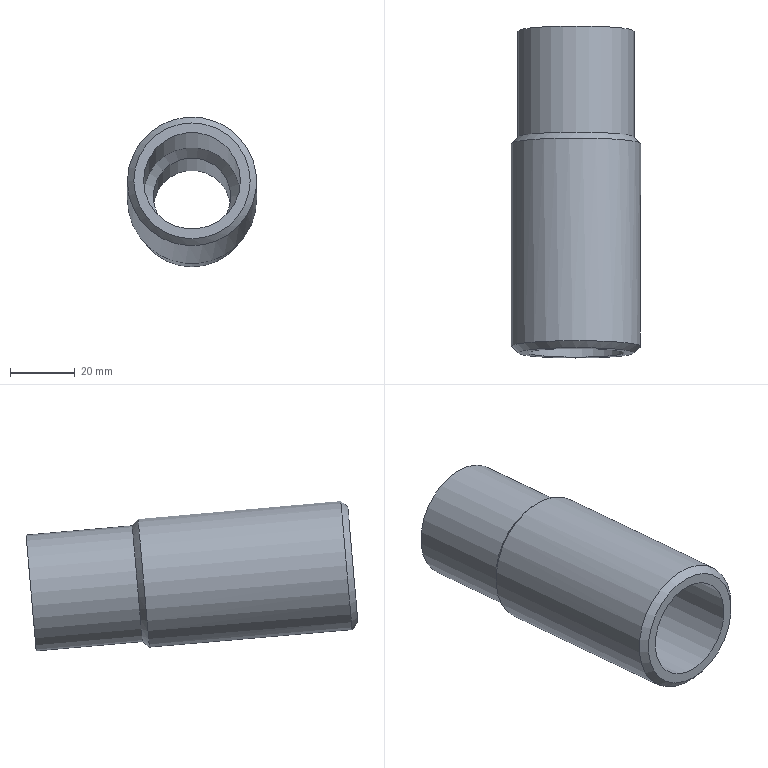Component | NX | HAND_NUT | 1 solid | 9 faces | box 40 x 102.76 x 46.4 mm | volume 58205 mm3 | cylinder 4 | cone 3 | plane 2 | commonest cylinder face diameters 40.005 x1 36.005 x1 30.006 x1 24.008 x1
STEP:
#1=CARTESIAN_POINT('',(0.,0.,0.));
#2=DIRECTION('',(0.,0.,1.));
#3=DIRECTION('',(1.,0.,0.));
#4=AXIS2_PLACEMENT_3D('',#1,#2,#3);
#5=CARTESIAN_POINT('',(323.937,425.208,3.169));
#6=VERTEX_POINT('',#5);
#7=CARTESIAN_POINT('',(335.941,425.208,3.169));
#8=DIRECTION('',(0.,0.9962,-0.08716));
#9=DIRECTION('',(-1.,0.,0.));
#10=AXIS2_PLACEMENT_3D('',#7,#8,#9);
#11=CIRCLE('',#10,12.004);
#12=CARTESIAN_POINT('',(353.941,425.235,3.474));
#13=DIRECTION('',(0.,-0.9962,0.08716));
#14=DIRECTION('',(1.,0.,0.));
#15=AXIS2_PLACEMENT_3D('',#12,#13,#14);
#16=PLANE('',#15);
#17=CARTESIAN_POINT('',(-30.004,-0.3063));
#18=CARTESIAN_POINT('',(-30.004,20.485));
#19=CARTESIAN_POINT('',(-11.998,10.089));
#20=CARTESIAN_POINT('',(6.008,-0.3063));
#21=CARTESIAN_POINT('',(-11.998,-10.702));
#22=CARTESIAN_POINT('',(-30.004,-21.098));
#23=CARTESIAN_POINT('',(-30.004,-0.3063));
#24=(BOUNDED_CURVE()B_SPLINE_CURVE(2,(#17,#18,#19,#20,#21,#22,#23),.UNSPECIFIED.,.T.,.F.)B_SPLINE_CURVE_WITH_KNOTS((1,2,2,2,2,1),(-2.094,0.,2.094,4.189,6.283,8.378),.UNSPECIFIED.)CURVE()GEOMETRIC_REPRESENTATION_ITEM()RATIONAL_B_SPLINE_CURVE((1.,0.5,1.,0.5,1.,0.5,1.))REPRESENTATION_ITEM(''));
#25=(GEOMETRIC_REPRESENTATION_CONTEXT(2)PARAMETRIC_REPRESENTATION_CONTEXT()REPRESENTATION_CONTEXT('',''));
#26=DEFINITIONAL_REPRESENTATION('',(#24),#25);
#27=PCURVE('',#16,#26);
#28=CARTESIAN_POINT('',(335.941,425.208,3.169));
#29=DIRECTION('',(0.,0.9962,-0.08716));
#30=DIRECTION('',(-1.,0.,0.));
#31=AXIS2_PLACEMENT_3D('',#28,#29,#30);
#32=CYLINDRICAL_SURFACE('',#31,12.004);
#33=CARTESIAN_POINT('',(0.,0.));
#34=DIRECTION('',(1.,0.));
#35=VECTOR('',#34,1.);
#36=LINE('',#33,#35);
#37=(GEOMETRIC_REPRESENTATION_CONTEXT(2)PARAMETRIC_REPRESENTATION_CONTEXT()REPRESENTATION_CONTEXT('',''));
#38=DEFINITIONAL_REPRESENTATION('',(#36),#37);
#39=PCURVE('',#32,#38);
#40=SURFACE_CURVE('',#11,(#27,#39),.PCURVE_S1.);
#41=EDGE_CURVE('',#6,#6,#40,.T.);
#42=ORIENTED_EDGE('',*,*,#41,.F.);
#43=EDGE_LOOP('',(#42));
#44=FACE_BOUND('',#43,.T.);
#45=CARTESIAN_POINT('',(317.939,425.208,3.169));
#46=VERTEX_POINT('',#45);
#47=CARTESIAN_POINT('',(335.941,425.208,3.169));
#48=DIRECTION('',(0.,0.9962,-0.08716));
#49=DIRECTION('',(-1.,0.,0.));
#50=AXIS2_PLACEMENT_3D('',#47,#48,#49);
#51=CIRCLE('',#50,18.003);
#52=CARTESIAN_POINT('',(-36.003,-0.3063));
#53=CARTESIAN_POINT('',(-36.003,30.875));
#54=CARTESIAN_POINT('',(-8.999,15.284));
#55=CARTESIAN_POINT('',(18.005,-0.3063));
#56=CARTESIAN_POINT('',(-8.999,-15.897));
#57=CARTESIAN_POINT('',(-36.003,-31.488));
#58=CARTESIAN_POINT('',(-36.003,-0.3063));
#59=(BOUNDED_CURVE()B_SPLINE_CURVE(2,(#52,#53,#54,#55,#56,#57,#58),.UNSPECIFIED.,.T.,.F.)B_SPLINE_CURVE_WITH_KNOTS((1,2,2,2,2,1),(-2.094,0.,2.094,4.189,6.283,8.378),.UNSPECIFIED.)CURVE()GEOMETRIC_REPRESENTATION_ITEM()RATIONAL_B_SPLINE_CURVE((1.,0.5,1.,0.5,1.,0.5,1.))REPRESENTATION_ITEM(''));
#60=(GEOMETRIC_REPRESENTATION_CONTEXT(2)PARAMETRIC_REPRESENTATION_CONTEXT()REPRESENTATION_CONTEXT('',''));
#61=DEFINITIONAL_REPRESENTATION('',(#59),#60);
#62=PCURVE('',#16,#61);
#63=CARTESIAN_POINT('',(335.941,367.621,8.207));
#64=DIRECTION('',(0.,0.9962,-0.08716));
#65=DIRECTION('',(-1.,0.,0.));
#66=AXIS2_PLACEMENT_3D('',#63,#64,#65);
#67=CYLINDRICAL_SURFACE('',#66,18.003);
#68=CARTESIAN_POINT('',(0.,57.808));
#69=DIRECTION('',(1.,0.));
#70=VECTOR('',#69,1.);
#71=LINE('',#68,#70);
#72=(GEOMETRIC_REPRESENTATION_CONTEXT(2)PARAMETRIC_REPRESENTATION_CONTEXT()REPRESENTATION_CONTEXT('',''));
#73=DEFINITIONAL_REPRESENTATION('',(#71),#72);
#74=PCURVE('',#67,#73);
#75=SURFACE_CURVE('',#51,(#62,#74),.PCURVE_S1.);
#76=EDGE_CURVE('',#46,#46,#75,.T.);
#77=ORIENTED_EDGE('',*,*,#76,.T.);
#78=EDGE_LOOP('',(#77));
#79=FACE_BOUND('',#78,.T.);
#80=ADVANCED_FACE('',(#44,#79),#16,.F.);
#81=CARTESIAN_POINT('',(317.939,325.589,11.884));
#82=VERTEX_POINT('',#81);
#83=CARTESIAN_POINT('',(335.941,325.589,11.884));
#84=DIRECTION('',(0.,-0.9962,0.08716));
#85=DIRECTION('',(-1.,0.,0.));
#86=AXIS2_PLACEMENT_3D('',#83,#84,#85);
#87=CIRCLE('',#86,18.002);
#88=CARTESIAN_POINT('',(335.941,325.616,12.189));
#89=DIRECTION('',(0.,0.9962,-0.08716));
#90=DIRECTION('',(-1.,0.,0.));
#91=AXIS2_PLACEMENT_3D('',#88,#89,#90);
#92=PLANE('',#91);
#93=CARTESIAN_POINT('',(18.002,-0.3063));
#94=CARTESIAN_POINT('',(18.002,-31.487));
#95=CARTESIAN_POINT('',(-9.001,-15.897));
#96=CARTESIAN_POINT('',(-36.005,-0.3063));
#97=CARTESIAN_POINT('',(-9.001,15.284));
#98=CARTESIAN_POINT('',(18.002,30.875));
#99=CARTESIAN_POINT('',(18.002,-0.3063));
#100=(BOUNDED_CURVE()B_SPLINE_CURVE(2,(#93,#94,#95,#96,#97,#98,#99),.UNSPECIFIED.,.T.,.F.)B_SPLINE_CURVE_WITH_KNOTS((1,2,2,2,2,1),(-2.094,0.,2.094,4.189,6.283,8.378),.UNSPECIFIED.)CURVE()GEOMETRIC_REPRESENTATION_ITEM()RATIONAL_B_SPLINE_CURVE((1.,0.5,1.,0.5,1.,0.5,1.))REPRESENTATION_ITEM(''));
#101=(GEOMETRIC_REPRESENTATION_CONTEXT(2)PARAMETRIC_REPRESENTATION_CONTEXT()REPRESENTATION_CONTEXT('',''));
#102=DEFINITIONAL_REPRESENTATION('',(#100),#101);
#103=PCURVE('',#92,#102);
#104=CARTESIAN_POINT('',(335.941,327.581,11.71));
#105=DIRECTION('',(0.,0.9962,-0.08716));
#106=DIRECTION('',(-1.,0.,0.));
#107=AXIS2_PLACEMENT_3D('',#104,#105,#106);
#108=CONICAL_SURFACE('',#107,20.002,0.7854);
#109=CARTESIAN_POINT('',(6.283,-2.));
#110=DIRECTION('',(-1.,0.));
#111=VECTOR('',#110,1.);
#112=LINE('',#109,#111);
#113=(GEOMETRIC_REPRESENTATION_CONTEXT(2)PARAMETRIC_REPRESENTATION_CONTEXT()REPRESENTATION_CONTEXT('',''));
#114=DEFINITIONAL_REPRESENTATION('',(#112),#113);
#115=PCURVE('',#108,#114);
#116=SURFACE_CURVE('',#87,(#103,#115),.PCURVE_S1.);
#117=EDGE_CURVE('',#82,#82,#116,.T.);
#118=ORIENTED_EDGE('',*,*,#117,.T.);
#119=EDGE_LOOP('',(#118));
#120=FACE_BOUND('',#119,.T.);
#121=CARTESIAN_POINT('',(320.938,325.589,11.884));
#122=VERTEX_POINT('',#121);
#123=CARTESIAN_POINT('',(335.941,325.589,11.884));
#124=DIRECTION('',(0.,0.9962,-0.08716));
#125=DIRECTION('',(-1.,0.,0.));
#126=AXIS2_PLACEMENT_3D('',#123,#124,#125);
#127=CIRCLE('',#126,15.003);
#128=CARTESIAN_POINT('',(0.,-0.3063));
#129=DIRECTION('',(1.,0.));
#130=AXIS2_PLACEMENT_2D('',#128,#129);
#131=CIRCLE('',#130,15.003);
#132=(GEOMETRIC_REPRESENTATION_CONTEXT(2)PARAMETRIC_REPRESENTATION_CONTEXT()REPRESENTATION_CONTEXT('',''));
#133=DEFINITIONAL_REPRESENTATION('',(#131),#132);
#134=PCURVE('',#92,#133);
#135=CARTESIAN_POINT('',(335.941,425.208,3.169));
#136=DIRECTION('',(0.,0.9962,-0.08716));
#137=DIRECTION('',(-1.,0.,0.));
#138=AXIS2_PLACEMENT_3D('',#135,#136,#137);
#139=CYLINDRICAL_SURFACE('',#138,15.003);
#140=CARTESIAN_POINT('',(0.,-100.));
#141=DIRECTION('',(1.,0.));
#142=VECTOR('',#141,1.);
#143=LINE('',#140,#142);
#144=(GEOMETRIC_REPRESENTATION_CONTEXT(2)PARAMETRIC_REPRESENTATION_CONTEXT()REPRESENTATION_CONTEXT('',''));
#145=DEFINITIONAL_REPRESENTATION('',(#143),#144);
#146=PCURVE('',#139,#145);
#147=SURFACE_CURVE('',#127,(#134,#146),.PCURVE_S1.);
#148=EDGE_CURVE('',#122,#122,#147,.T.);
#149=ORIENTED_EDGE('',*,*,#148,.T.);
#150=EDGE_LOOP('',(#149));
#151=FACE_BOUND('',#150,.T.);
#152=ADVANCED_FACE('',(#120,#151),#92,.F.);
#153=CARTESIAN_POINT('',(355.943,390.342,6.219));
#154=VERTEX_POINT('',#153);
#155=CARTESIAN_POINT('',(315.939,390.342,6.219));
#156=VERTEX_POINT('',#155);
#157=CARTESIAN_POINT('',(335.941,390.342,6.219));
#158=DIRECTION('',(0.,-0.9962,0.08716));
#159=DIRECTION('',(1.,0.,0.));
#160=AXIS2_PLACEMENT_3D('',#157,#158,#159);
#161=CIRCLE('',#160,20.002);
#162=CARTESIAN_POINT('',(335.941,367.621,8.207));
#163=DIRECTION('',(0.,0.9962,-0.08716));
#164=DIRECTION('',(-1.,0.,0.));
#165=AXIS2_PLACEMENT_3D('',#162,#163,#164);
#166=CYLINDRICAL_SURFACE('',#165,20.002);
#167=CARTESIAN_POINT('',(3.142,22.808));
#168=DIRECTION('',(-1.,0.));
#169=VECTOR('',#168,1.);
#170=LINE('',#167,#169);
#171=(GEOMETRIC_REPRESENTATION_CONTEXT(2)PARAMETRIC_REPRESENTATION_CONTEXT()REPRESENTATION_CONTEXT('',''));
#172=DEFINITIONAL_REPRESENTATION('',(#170),#171);
#173=PCURVE('',#166,#172);
#174=CARTESIAN_POINT('',(335.941,392.334,6.045));
#175=DIRECTION('',(0.,-0.9962,0.08716));
#176=DIRECTION('',(1.,0.,0.));
#177=AXIS2_PLACEMENT_3D('',#174,#175,#176);
#178=CONICAL_SURFACE('',#177,18.003,0.7854);
#179=CARTESIAN_POINT('',(0.,2.));
#180=DIRECTION('',(1.,0.));
#181=VECTOR('',#180,1.);
#182=LINE('',#179,#181);
#183=(GEOMETRIC_REPRESENTATION_CONTEXT(2)PARAMETRIC_REPRESENTATION_CONTEXT()REPRESENTATION_CONTEXT('',''));
#184=DEFINITIONAL_REPRESENTATION('',(#182),#183);
#185=PCURVE('',#178,#184);
#186=SURFACE_CURVE('',#161,(#173,#185),.PCURVE_S1.);
#187=EDGE_CURVE('',#154,#156,#186,.T.);
#188=ORIENTED_EDGE('',*,*,#187,.T.);
#189=CARTESIAN_POINT('',(315.939,327.581,11.71));
#190=VERTEX_POINT('',#189);
#191=CARTESIAN_POINT('',(315.939,327.581,11.71));
#192=CARTESIAN_POINT('',(315.939,390.342,6.219));
#193=B_SPLINE_CURVE_WITH_KNOTS('',1,(#191,#192),.UNSPECIFIED.,.F.,.F.,(2,2),(-40.192,22.808),.PIECEWISE_BEZIER_KNOTS.);
#194=CARTESIAN_POINT('',(0.,0.));
#195=DIRECTION('',(0.,1.));
#196=VECTOR('',#195,1.);
#197=LINE('',#194,#196);
#198=(GEOMETRIC_REPRESENTATION_CONTEXT(2)PARAMETRIC_REPRESENTATION_CONTEXT()REPRESENTATION_CONTEXT('',''));
#199=DEFINITIONAL_REPRESENTATION('',(#197),#198);
#200=PCURVE('',#166,#199);
#201=CARTESIAN_POINT('',(6.283,0.));
#202=DIRECTION('',(0.,1.));
#203=VECTOR('',#202,1.);
#204=LINE('',#201,#203);
#205=(GEOMETRIC_REPRESENTATION_CONTEXT(2)PARAMETRIC_REPRESENTATION_CONTEXT()REPRESENTATION_CONTEXT('',''));
#206=DEFINITIONAL_REPRESENTATION('',(#204),#205);
#207=PCURVE('',#166,#206);
#208=SEAM_CURVE('',#193,(#200,#207),.PCURVE_S1.);
#209=EDGE_CURVE('',#190,#156,#208,.T.);
#210=ORIENTED_EDGE('',*,*,#209,.F.);
#211=CARTESIAN_POINT('',(335.941,327.581,11.71));
#212=DIRECTION('',(0.,0.9962,-0.08716));
#213=DIRECTION('',(-1.,0.,0.));
#214=AXIS2_PLACEMENT_3D('',#211,#212,#213);
#215=CIRCLE('',#214,20.002);
#216=CARTESIAN_POINT('',(0.,-40.192));
#217=DIRECTION('',(1.,0.));
#218=VECTOR('',#217,1.);
#219=LINE('',#216,#218);
#220=(GEOMETRIC_REPRESENTATION_CONTEXT(2)PARAMETRIC_REPRESENTATION_CONTEXT()REPRESENTATION_CONTEXT('',''));
#221=DEFINITIONAL_REPRESENTATION('',(#219),#220);
#222=PCURVE('',#166,#221);
#223=CARTESIAN_POINT('',(0.,0.));
#224=DIRECTION('',(1.,0.));
#225=VECTOR('',#224,1.);
#226=LINE('',#223,#225);
#227=(GEOMETRIC_REPRESENTATION_CONTEXT(2)PARAMETRIC_REPRESENTATION_CONTEXT()REPRESENTATION_CONTEXT('',''));
#228=DEFINITIONAL_REPRESENTATION('',(#226),#227);
#229=PCURVE('',#108,#228);
#230=SURFACE_CURVE('',#215,(#222,#229),.PCURVE_S1.);
#231=EDGE_CURVE('',#190,#190,#230,.T.);
#232=ORIENTED_EDGE('',*,*,#231,.T.);
#233=ORIENTED_EDGE('',*,*,#209,.T.);
#234=CARTESIAN_POINT('',(335.941,390.342,6.219));
#235=DIRECTION('',(0.,-0.9962,0.08716));
#236=DIRECTION('',(1.,0.,0.));
#237=AXIS2_PLACEMENT_3D('',#234,#235,#236);
#238=CIRCLE('',#237,20.002);
#239=CARTESIAN_POINT('',(9.425,22.808));
#240=DIRECTION('',(-1.,0.));
#241=VECTOR('',#240,1.);
#242=LINE('',#239,#241);
#243=(GEOMETRIC_REPRESENTATION_CONTEXT(2)PARAMETRIC_REPRESENTATION_CONTEXT()REPRESENTATION_CONTEXT('',''));
#244=DEFINITIONAL_REPRESENTATION('',(#242),#243);
#245=PCURVE('',#166,#244);
#246=CARTESIAN_POINT('',(0.,2.));
#247=DIRECTION('',(1.,0.));
#248=VECTOR('',#247,1.);
#249=LINE('',#246,#248);
#250=(GEOMETRIC_REPRESENTATION_CONTEXT(2)PARAMETRIC_REPRESENTATION_CONTEXT()REPRESENTATION_CONTEXT('',''));
#251=DEFINITIONAL_REPRESENTATION('',(#249),#250);
#252=PCURVE('',#178,#251);
#253=SURFACE_CURVE('',#238,(#245,#252),.PCURVE_S1.);
#254=EDGE_CURVE('',#156,#154,#253,.T.);
#255=ORIENTED_EDGE('',*,*,#254,.T.);
#256=EDGE_LOOP('',(#188,#210,#232,#233,#255));
#257=FACE_BOUND('',#256,.T.);
#258=ADVANCED_FACE('',(#257),#166,.T.);
#259=CARTESIAN_POINT('',(353.944,392.334,6.045));
#260=VERTEX_POINT('',#259);
#261=CARTESIAN_POINT('',(317.939,392.334,6.045));
#262=VERTEX_POINT('',#261);
#263=CARTESIAN_POINT('',(335.941,392.334,6.045));
#264=DIRECTION('',(0.,0.9962,-0.08716));
#265=DIRECTION('',(1.,0.,0.));
#266=AXIS2_PLACEMENT_3D('',#263,#264,#265);
#267=CIRCLE('',#266,18.003);
#268=CARTESIAN_POINT('',(3.142,24.808));
#269=DIRECTION('',(1.,0.));
#270=VECTOR('',#269,1.);
#271=LINE('',#268,#270);
#272=(GEOMETRIC_REPRESENTATION_CONTEXT(2)PARAMETRIC_REPRESENTATION_CONTEXT()REPRESENTATION_CONTEXT('',''));
#273=DEFINITIONAL_REPRESENTATION('',(#271),#272);
#274=PCURVE('',#67,#273);
#275=CARTESIAN_POINT('',(6.283,-0.));
#276=DIRECTION('',(-1.,0.));
#277=VECTOR('',#276,1.);
#278=LINE('',#275,#277);
#279=(GEOMETRIC_REPRESENTATION_CONTEXT(2)PARAMETRIC_REPRESENTATION_CONTEXT()REPRESENTATION_CONTEXT('',''));
#280=DEFINITIONAL_REPRESENTATION('',(#278),#279);
#281=PCURVE('',#178,#280);
#282=SURFACE_CURVE('',#267,(#274,#281),.PCURVE_S1.);
#283=EDGE_CURVE('',#260,#262,#282,.T.);
#284=ORIENTED_EDGE('',*,*,#283,.T.);
#285=CARTESIAN_POINT('',(317.939,392.334,6.045));
#286=CARTESIAN_POINT('',(317.939,425.208,3.169));
#287=B_SPLINE_CURVE_WITH_KNOTS('',1,(#285,#286),.UNSPECIFIED.,.F.,.F.,(2,2),(24.808,57.808),.PIECEWISE_BEZIER_KNOTS.);
#288=CARTESIAN_POINT('',(6.283,0.));
#289=DIRECTION('',(0.,1.));
#290=VECTOR('',#289,1.);
#291=LINE('',#288,#290);
#292=(GEOMETRIC_REPRESENTATION_CONTEXT(2)PARAMETRIC_REPRESENTATION_CONTEXT()REPRESENTATION_CONTEXT('',''));
#293=DEFINITIONAL_REPRESENTATION('',(#291),#292);
#294=PCURVE('',#67,#293);
#295=CARTESIAN_POINT('',(0.,0.));
#296=DIRECTION('',(0.,1.));
#297=VECTOR('',#296,1.);
#298=LINE('',#295,#297);
#299=(GEOMETRIC_REPRESENTATION_CONTEXT(2)PARAMETRIC_REPRESENTATION_CONTEXT()REPRESENTATION_CONTEXT('',''));
#300=DEFINITIONAL_REPRESENTATION('',(#298),#299);
#301=PCURVE('',#67,#300);
#302=SEAM_CURVE('',#287,(#294,#301),.PCURVE_S1.);
#303=EDGE_CURVE('',#262,#46,#302,.T.);
#304=ORIENTED_EDGE('',*,*,#303,.T.);
#305=ORIENTED_EDGE('',*,*,#76,.F.);
#306=ORIENTED_EDGE('',*,*,#303,.F.);
#307=CARTESIAN_POINT('',(335.941,392.334,6.045));
#308=DIRECTION('',(0.,0.9962,-0.08716));
#309=DIRECTION('',(1.,0.,0.));
#310=AXIS2_PLACEMENT_3D('',#307,#308,#309);
#311=CIRCLE('',#310,18.003);
#312=CARTESIAN_POINT('',(-3.142,24.808));
#313=DIRECTION('',(1.,0.));
#314=VECTOR('',#313,1.);
#315=LINE('',#312,#314);
#316=(GEOMETRIC_REPRESENTATION_CONTEXT(2)PARAMETRIC_REPRESENTATION_CONTEXT()REPRESENTATION_CONTEXT('',''));
#317=DEFINITIONAL_REPRESENTATION('',(#315),#316);
#318=PCURVE('',#67,#317);
#319=CARTESIAN_POINT('',(6.283,-0.));
#320=DIRECTION('',(-1.,0.));
#321=VECTOR('',#320,1.);
#322=LINE('',#319,#321);
#323=(GEOMETRIC_REPRESENTATION_CONTEXT(2)PARAMETRIC_REPRESENTATION_CONTEXT()REPRESENTATION_CONTEXT('',''));
#324=DEFINITIONAL_REPRESENTATION('',(#322),#323);
#325=PCURVE('',#178,#324);
#326=SURFACE_CURVE('',#311,(#318,#325),.PCURVE_S1.);
#327=EDGE_CURVE('',#262,#260,#326,.T.);
#328=ORIENTED_EDGE('',*,*,#327,.T.);
#329=EDGE_LOOP('',(#284,#304,#305,#306,#328));
#330=FACE_BOUND('',#329,.T.);
#331=ADVANCED_FACE('',(#330),#67,.T.);
#332=CARTESIAN_POINT('',(320.938,378.387,7.265));
#333=VERTEX_POINT('',#332);
#334=CARTESIAN_POINT('',(350.944,378.387,7.265));
#335=VERTEX_POINT('',#334);
#336=CARTESIAN_POINT('',(335.941,378.387,7.265));
#337=DIRECTION('',(0.,0.9962,-0.08716));
#338=DIRECTION('',(1.,0.,0.));
#339=AXIS2_PLACEMENT_3D('',#336,#337,#338);
#340=CIRCLE('',#339,15.003);
#341=CARTESIAN_POINT('',(-3.142,-47.));
#342=DIRECTION('',(1.,0.));
#343=VECTOR('',#342,1.);
#344=LINE('',#341,#343);
#345=(GEOMETRIC_REPRESENTATION_CONTEXT(2)PARAMETRIC_REPRESENTATION_CONTEXT()REPRESENTATION_CONTEXT('',''));
#346=DEFINITIONAL_REPRESENTATION('',(#344),#345);
#347=PCURVE('',#139,#346);
#348=CARTESIAN_POINT('',(335.941,382.372,6.916));
#349=DIRECTION('',(0.,-0.9962,0.08716));
#350=DIRECTION('',(1.,-0.,-0.));
#351=AXIS2_PLACEMENT_3D('',#348,#349,#350);
#352=CONICAL_SURFACE('',#351,11.003,0.7854);
#353=CARTESIAN_POINT('',(6.283,4.));
#354=DIRECTION('',(-1.,0.));
#355=VECTOR('',#354,1.);
#356=LINE('',#353,#355);
#357=(GEOMETRIC_REPRESENTATION_CONTEXT(2)PARAMETRIC_REPRESENTATION_CONTEXT()REPRESENTATION_CONTEXT('',''));
#358=DEFINITIONAL_REPRESENTATION('',(#356),#357);
#359=PCURVE('',#352,#358);
#360=SURFACE_CURVE('',#340,(#347,#359),.PCURVE_S1.);
#361=EDGE_CURVE('',#333,#335,#360,.T.);
#362=ORIENTED_EDGE('',*,*,#361,.F.);
#363=CARTESIAN_POINT('',(320.938,325.589,11.884));
#364=CARTESIAN_POINT('',(320.938,378.387,7.265));
#365=B_SPLINE_CURVE_WITH_KNOTS('',1,(#363,#364),.UNSPECIFIED.,.F.,.F.,(2,2),(-100.,-47.),.PIECEWISE_BEZIER_KNOTS.);
#366=CARTESIAN_POINT('',(0.,0.));
#367=DIRECTION('',(0.,1.));
#368=VECTOR('',#367,1.);
#369=LINE('',#366,#368);
#370=(GEOMETRIC_REPRESENTATION_CONTEXT(2)PARAMETRIC_REPRESENTATION_CONTEXT()REPRESENTATION_CONTEXT('',''));
#371=DEFINITIONAL_REPRESENTATION('',(#369),#370);
#372=PCURVE('',#139,#371);
#373=CARTESIAN_POINT('',(6.283,0.));
#374=DIRECTION('',(0.,1.));
#375=VECTOR('',#374,1.);
#376=LINE('',#373,#375);
#377=(GEOMETRIC_REPRESENTATION_CONTEXT(2)PARAMETRIC_REPRESENTATION_CONTEXT()REPRESENTATION_CONTEXT('',''));
#378=DEFINITIONAL_REPRESENTATION('',(#376),#377);
#379=PCURVE('',#139,#378);
#380=SEAM_CURVE('',#365,(#372,#379),.PCURVE_S1.);
#381=EDGE_CURVE('',#122,#333,#380,.T.);
#382=ORIENTED_EDGE('',*,*,#381,.F.);
#383=ORIENTED_EDGE('',*,*,#148,.T.);
#384=ORIENTED_EDGE('',*,*,#381,.T.);
#385=CARTESIAN_POINT('',(335.941,378.387,7.265));
#386=DIRECTION('',(0.,0.9962,-0.08716));
#387=DIRECTION('',(1.,0.,0.));
#388=AXIS2_PLACEMENT_3D('',#385,#386,#387);
#389=CIRCLE('',#388,15.003);
#390=CARTESIAN_POINT('',(3.142,-47.));
#391=DIRECTION('',(1.,0.));
#392=VECTOR('',#391,1.);
#393=LINE('',#390,#392);
#394=(GEOMETRIC_REPRESENTATION_CONTEXT(2)PARAMETRIC_REPRESENTATION_CONTEXT()REPRESENTATION_CONTEXT('',''));
#395=DEFINITIONAL_REPRESENTATION('',(#393),#394);
#396=PCURVE('',#139,#395);
#397=CARTESIAN_POINT('',(6.283,4.));
#398=DIRECTION('',(-1.,0.));
#399=VECTOR('',#398,1.);
#400=LINE('',#397,#399);
#401=(GEOMETRIC_REPRESENTATION_CONTEXT(2)PARAMETRIC_REPRESENTATION_CONTEXT()REPRESENTATION_CONTEXT('',''));
#402=DEFINITIONAL_REPRESENTATION('',(#400),#401);
#403=PCURVE('',#352,#402);
#404=SURFACE_CURVE('',#389,(#396,#403),.PCURVE_S1.);
#405=EDGE_CURVE('',#335,#333,#404,.T.);
#406=ORIENTED_EDGE('',*,*,#405,.F.);
#407=EDGE_LOOP('',(#362,#382,#383,#384,#406));
#408=FACE_BOUND('',#407,.F.);
#409=ADVANCED_FACE('',(#408),#139,.F.);
#410=CARTESIAN_POINT('',(323.937,381.375,7.004));
#411=VERTEX_POINT('',#410);
#412=CARTESIAN_POINT('',(347.945,381.375,7.004));
#413=VERTEX_POINT('',#412);
#414=CARTESIAN_POINT('',(335.941,381.375,7.004));
#415=DIRECTION('',(0.,-0.9962,0.08716));
#416=DIRECTION('',(1.,0.,0.));
#417=AXIS2_PLACEMENT_3D('',#414,#415,#416);
#418=CIRCLE('',#417,12.004);
#419=CARTESIAN_POINT('',(9.425,-44.001));
#420=DIRECTION('',(-1.,0.));
#421=VECTOR('',#420,1.);
#422=LINE('',#419,#421);
#423=(GEOMETRIC_REPRESENTATION_CONTEXT(2)PARAMETRIC_REPRESENTATION_CONTEXT()REPRESENTATION_CONTEXT('',''));
#424=DEFINITIONAL_REPRESENTATION('',(#422),#423);
#425=PCURVE('',#32,#424);
#426=CARTESIAN_POINT('',(0.,1.001));
#427=DIRECTION('',(1.,0.));
#428=VECTOR('',#427,1.);
#429=LINE('',#426,#428);
#430=(GEOMETRIC_REPRESENTATION_CONTEXT(2)PARAMETRIC_REPRESENTATION_CONTEXT()REPRESENTATION_CONTEXT('',''));
#431=DEFINITIONAL_REPRESENTATION('',(#429),#430);
#432=PCURVE('',#352,#431);
#433=SURFACE_CURVE('',#418,(#425,#432),.PCURVE_S1.);
#434=EDGE_CURVE('',#411,#413,#433,.T.);
#435=ORIENTED_EDGE('',*,*,#434,.F.);
#436=CARTESIAN_POINT('',(323.937,381.375,7.004));
#437=CARTESIAN_POINT('',(323.937,425.208,3.169));
#438=B_SPLINE_CURVE_WITH_KNOTS('',1,(#436,#437),.UNSPECIFIED.,.F.,.F.,(2,2),(-44.001,0.),.PIECEWISE_BEZIER_KNOTS.);
#439=CARTESIAN_POINT('',(6.283,0.));
#440=DIRECTION('',(0.,1.));
#441=VECTOR('',#440,1.);
#442=LINE('',#439,#441);
#443=(GEOMETRIC_REPRESENTATION_CONTEXT(2)PARAMETRIC_REPRESENTATION_CONTEXT()REPRESENTATION_CONTEXT('',''));
#444=DEFINITIONAL_REPRESENTATION('',(#442),#443);
#445=PCURVE('',#32,#444);
#446=CARTESIAN_POINT('',(0.,0.));
#447=DIRECTION('',(0.,1.));
#448=VECTOR('',#447,1.);
#449=LINE('',#446,#448);
#450=(GEOMETRIC_REPRESENTATION_CONTEXT(2)PARAMETRIC_REPRESENTATION_CONTEXT()REPRESENTATION_CONTEXT('',''));
#451=DEFINITIONAL_REPRESENTATION('',(#449),#450);
#452=PCURVE('',#32,#451);
#453=SEAM_CURVE('',#438,(#445,#452),.PCURVE_S1.);
#454=EDGE_CURVE('',#411,#6,#453,.T.);
#455=ORIENTED_EDGE('',*,*,#454,.T.);
#456=ORIENTED_EDGE('',*,*,#41,.F.);
#457=ORIENTED_EDGE('',*,*,#454,.F.);
#458=CARTESIAN_POINT('',(335.941,381.375,7.004));
#459=DIRECTION('',(0.,-0.9962,0.08716));
#460=DIRECTION('',(1.,0.,0.));
#461=AXIS2_PLACEMENT_3D('',#458,#459,#460);
#462=CIRCLE('',#461,12.004);
#463=CARTESIAN_POINT('',(3.142,-44.001));
#464=DIRECTION('',(-1.,0.));
#465=VECTOR('',#464,1.);
#466=LINE('',#463,#465);
#467=(GEOMETRIC_REPRESENTATION_CONTEXT(2)PARAMETRIC_REPRESENTATION_CONTEXT()REPRESENTATION_CONTEXT('',''));
#468=DEFINITIONAL_REPRESENTATION('',(#466),#467);
#469=PCURVE('',#32,#468);
#470=CARTESIAN_POINT('',(0.,1.001));
#471=DIRECTION('',(1.,0.));
#472=VECTOR('',#471,1.);
#473=LINE('',#470,#472);
#474=(GEOMETRIC_REPRESENTATION_CONTEXT(2)PARAMETRIC_REPRESENTATION_CONTEXT()REPRESENTATION_CONTEXT('',''));
#475=DEFINITIONAL_REPRESENTATION('',(#473),#474);
#476=PCURVE('',#352,#475);
#477=SURFACE_CURVE('',#462,(#469,#476),.PCURVE_S1.);
#478=EDGE_CURVE('',#413,#411,#477,.T.);
#479=ORIENTED_EDGE('',*,*,#478,.F.);
#480=EDGE_LOOP('',(#435,#455,#456,#457,#479));
#481=FACE_BOUND('',#480,.F.);
#482=ADVANCED_FACE('',(#481),#32,.F.);
#483=ORIENTED_EDGE('',*,*,#361,.T.);
#484=CARTESIAN_POINT('',(347.945,381.375,7.004));
#485=CARTESIAN_POINT('',(350.944,378.387,7.265));
#486=B_SPLINE_CURVE_WITH_KNOTS('',1,(#484,#485),.UNSPECIFIED.,.F.,.F.,(2,2),(1.415,5.657),.PIECEWISE_BEZIER_KNOTS.);
#487=CARTESIAN_POINT('',(0.,0.));
#488=DIRECTION('',(0.,1.));
#489=VECTOR('',#488,1.);
#490=LINE('',#487,#489);
#491=(GEOMETRIC_REPRESENTATION_CONTEXT(2)PARAMETRIC_REPRESENTATION_CONTEXT()REPRESENTATION_CONTEXT('',''));
#492=DEFINITIONAL_REPRESENTATION('',(#490),#491);
#493=PCURVE('',#352,#492);
#494=CARTESIAN_POINT('',(6.283,0.));
#495=DIRECTION('',(0.,1.));
#496=VECTOR('',#495,1.);
#497=LINE('',#494,#496);
#498=(GEOMETRIC_REPRESENTATION_CONTEXT(2)PARAMETRIC_REPRESENTATION_CONTEXT()REPRESENTATION_CONTEXT('',''));
#499=DEFINITIONAL_REPRESENTATION('',(#497),#498);
#500=PCURVE('',#352,#499);
#501=SEAM_CURVE('',#486,(#493,#500),.PCURVE_S1.);
#502=EDGE_CURVE('',#413,#335,#501,.T.);
#503=ORIENTED_EDGE('',*,*,#502,.F.);
#504=ORIENTED_EDGE('',*,*,#478,.T.);
#505=ORIENTED_EDGE('',*,*,#434,.T.);
#506=ORIENTED_EDGE('',*,*,#502,.T.);
#507=ORIENTED_EDGE('',*,*,#405,.T.);
#508=EDGE_LOOP('',(#483,#503,#504,#505,#506,#507));
#509=FACE_BOUND('',#508,.F.);
#510=ADVANCED_FACE('',(#509),#352,.F.);
#511=ORIENTED_EDGE('',*,*,#117,.F.);
#512=CARTESIAN_POINT('',(317.939,325.589,11.884));
#513=CARTESIAN_POINT('',(315.939,327.581,11.71));
#514=B_SPLINE_CURVE_WITH_KNOTS('',1,(#512,#513),.UNSPECIFIED.,.F.,.F.,(2,2),(-2.828,0.),.PIECEWISE_BEZIER_KNOTS.);
#515=CARTESIAN_POINT('',(6.283,0.));
#516=DIRECTION('',(0.,1.));
#517=VECTOR('',#516,1.);
#518=LINE('',#515,#517);
#519=(GEOMETRIC_REPRESENTATION_CONTEXT(2)PARAMETRIC_REPRESENTATION_CONTEXT()REPRESENTATION_CONTEXT('',''));
#520=DEFINITIONAL_REPRESENTATION('',(#518),#519);
#521=PCURVE('',#108,#520);
#522=CARTESIAN_POINT('',(0.,0.));
#523=DIRECTION('',(0.,1.));
#524=VECTOR('',#523,1.);
#525=LINE('',#522,#524);
#526=(GEOMETRIC_REPRESENTATION_CONTEXT(2)PARAMETRIC_REPRESENTATION_CONTEXT()REPRESENTATION_CONTEXT('',''));
#527=DEFINITIONAL_REPRESENTATION('',(#525),#526);
#528=PCURVE('',#108,#527);
#529=SEAM_CURVE('',#514,(#521,#528),.PCURVE_S1.);
#530=EDGE_CURVE('',#82,#190,#529,.T.);
#531=ORIENTED_EDGE('',*,*,#530,.T.);
#532=ORIENTED_EDGE('',*,*,#231,.F.);
#533=ORIENTED_EDGE('',*,*,#530,.F.);
#534=EDGE_LOOP('',(#511,#531,#532,#533));
#535=FACE_BOUND('',#534,.T.);
#536=ADVANCED_FACE('',(#535),#108,.T.);
#537=ORIENTED_EDGE('',*,*,#187,.F.);
#538=CARTESIAN_POINT('',(353.944,392.334,6.045));
#539=CARTESIAN_POINT('',(355.943,390.342,6.219));
#540=B_SPLINE_CURVE_WITH_KNOTS('',1,(#538,#539),.UNSPECIFIED.,.F.,.F.,(2,2),(-0.,2.828),.PIECEWISE_BEZIER_KNOTS.);
#541=CARTESIAN_POINT('',(0.,0.));
#542=DIRECTION('',(0.,1.));
#543=VECTOR('',#542,1.);
#544=LINE('',#541,#543);
#545=(GEOMETRIC_REPRESENTATION_CONTEXT(2)PARAMETRIC_REPRESENTATION_CONTEXT()REPRESENTATION_CONTEXT('',''));
#546=DEFINITIONAL_REPRESENTATION('',(#544),#545);
#547=PCURVE('',#178,#546);
#548=CARTESIAN_POINT('',(6.283,0.));
#549=DIRECTION('',(0.,1.));
#550=VECTOR('',#549,1.);
#551=LINE('',#548,#550);
#552=(GEOMETRIC_REPRESENTATION_CONTEXT(2)PARAMETRIC_REPRESENTATION_CONTEXT()REPRESENTATION_CONTEXT('',''));
#553=DEFINITIONAL_REPRESENTATION('',(#551),#552);
#554=PCURVE('',#178,#553);
#555=SEAM_CURVE('',#540,(#547,#554),.PCURVE_S1.);
#556=EDGE_CURVE('',#260,#154,#555,.T.);
#557=ORIENTED_EDGE('',*,*,#556,.F.);
#558=ORIENTED_EDGE('',*,*,#327,.F.);
#559=ORIENTED_EDGE('',*,*,#283,.F.);
#560=ORIENTED_EDGE('',*,*,#556,.T.);
#561=ORIENTED_EDGE('',*,*,#254,.F.);
#562=EDGE_LOOP('',(#537,#557,#558,#559,#560,#561));
#563=FACE_BOUND('',#562,.T.);
#564=ADVANCED_FACE('',(#563),#178,.T.);
#565=CLOSED_SHELL('',(#80,#152,#258,#331,#409,#482,#510,#536,#564));
#566=MANIFOLD_SOLID_BREP('',#565);
#567=(LENGTH_UNIT()NAMED_UNIT(*)SI_UNIT(.MILLI.,.METRE.));
#568=UNCERTAINTY_MEASURE_WITH_UNIT(LENGTH_MEASURE(0.00001),#567,'','');
#569=(NAMED_UNIT(*)PLANE_ANGLE_UNIT()SI_UNIT($,.RADIAN.));
#570=(NAMED_UNIT(*)SI_UNIT($,.STERADIAN.)SOLID_ANGLE_UNIT());
#571=(GEOMETRIC_REPRESENTATION_CONTEXT(3)GLOBAL_UNCERTAINTY_ASSIGNED_CONTEXT((#568))GLOBAL_UNIT_ASSIGNED_CONTEXT((#567,#569,#570))REPRESENTATION_CONTEXT('',''));
#572=ADVANCED_BREP_SHAPE_REPRESENTATION('',(#4,#566),#571);